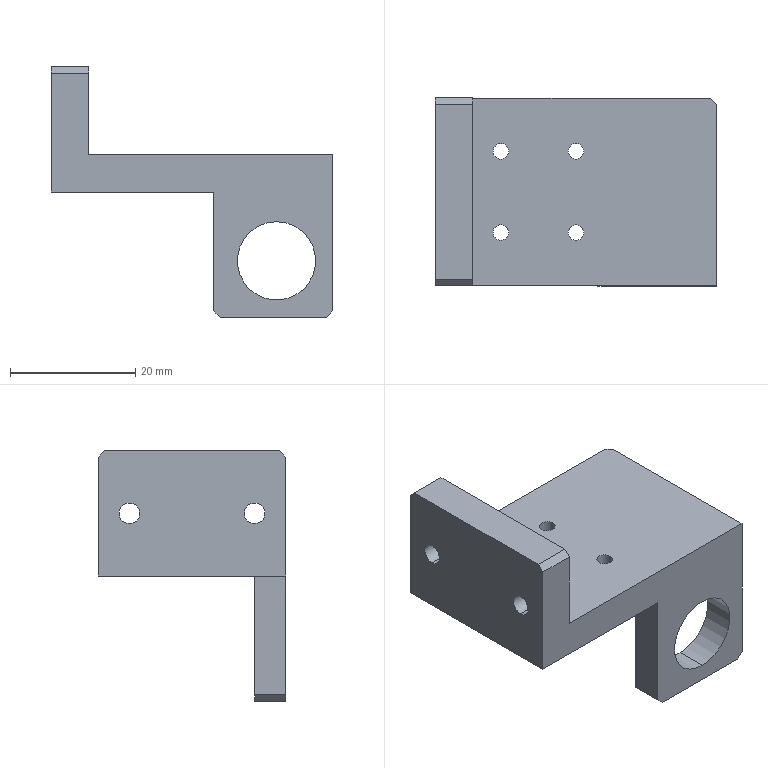Component | SolidWorks | F01AE00111-A5211-1 | 1 solid | 34 faces | box 45 x 30 x 40 mm | volume 11634 mm3 | cylinder 16 | plane 16 | cone 2 | commonest cylinder face diameters 2.5 x10 3.3 x4 12.5 x2
build123d program:
from build123d import *

# Parameters (mm, degrees)
SKETCH1_W             = 45
SKETCH1_H             = 30
BOSS_EXTRUDE1_DEPTH   = 3
SKETCH3_W             = 6
SKETCH3_H             = 30
BOSS_EXTRUDE3_DEPTH   = 14
M4_TAPPED_HOLE1_D     = 3.3
M4_TAPPED_HOLE1_DEPTH = 10.1
M4_TAPPED_HOLE1_TIP   = 0.9914
SKETCH9_W             = 19
SKETCH9_H             = 5
BOSS_EXTRUDE4_DEPTH   = 20
SKETCH10_R            = 6.25
CUT_EXTRUDE2_DEPTH    = 41.746
CHAMFER1_SIZE         = 1
SKETCH11_R            = 1.25
CUT_EXTRUDE3_DEPTH    = 38.513
M3_TAPPED_HOLE1_D     = 2.5
M3_TAPPED_HOLE1_DEPTH = 7.5
M3_TAPPED_HOLE1_TIP   = 0.7511


with BuildPart() as part:
    # Sketch1 → Boss-Extrude1 (new, symmetric)
    with BuildSketch(Plane.XY):
        Rectangle(SKETCH1_W, SKETCH1_H)
    extrude(amount=BOSS_EXTRUDE1_DEPTH, both=True)

    # Sketch3 → Boss-Extrude3 (add)
    with BuildSketch(Plane.XY.offset(3)):
        with Locations((-19.5, 0)):
            Rectangle(SKETCH3_W, SKETCH3_H)
    extrude(amount=BOSS_EXTRUDE3_DEPTH)

    # M4 Tapped Hole1
    with Locations(Plane.ZY.offset(22.5)):
        with Locations((7, -10), (7, 10)):
            Hole(M4_TAPPED_HOLE1_D / 2, depth=M4_TAPPED_HOLE1_DEPTH)
            with Locations((0, 0, -(M4_TAPPED_HOLE1_DEPTH + M4_TAPPED_HOLE1_TIP / 2))):  # 118° drill point
                Cone(0, M4_TAPPED_HOLE1_D / 2, M4_TAPPED_HOLE1_TIP, mode=Mode.SUBTRACT)

    # Sketch9 → Boss-Extrude4 (add)
    with BuildSketch(Plane(origin=(0, 0, -3), x_dir=(-1, 0, 0), z_dir=(0, 0, -1))):
        with Locations((-13, -12.5)):
            Rectangle(SKETCH9_W, SKETCH9_H)
    extrude(amount=BOSS_EXTRUDE4_DEPTH)

    # Sketch10 → Cut-Extrude2 (cut, through all)
    with BuildSketch(Plane(origin=(0, -10, 0), x_dir=(-1, 0, 0), z_dir=(0, 1, 0))):
        with Locations(Location((-13.5, -14, 0), (0, 0, 90))):
            Circle(SKETCH10_R)
    extrude(amount=-CUT_EXTRUDE2_DEPTH, mode=Mode.SUBTRACT)

    # Chamfer1
    chamfer1_edges = [part.edges().sort_by_distance(p)[0] for p in [
        (-19.5, -15, 17),
        (-19.5, 15, 17),
        (22.5, 15, 0),
        (22.5, -12.5, -23),
        (3.5, -12.5, -23),
    ]]
    chamfer(chamfer1_edges, length=CHAMFER1_SIZE)

    # Sketch11 → Cut-Extrude3 (cut, through all)
    with BuildSketch(Plane.XY.offset(3)):
        with Locations((-12, 6.5)):
            Circle(SKETCH11_R)
        with Locations((0, 6.5)):
            Circle(SKETCH11_R)
        with Locations((-12, -6.5)):
            Circle(SKETCH11_R)
        with Locations((0, -6.5)):
            Circle(SKETCH11_R)
    extrude(amount=-CUT_EXTRUDE3_DEPTH, mode=Mode.SUBTRACT)

    # M3 Tapped Hole1
    with Locations(Plane(origin=(0, 0, -23), x_dir=(-1, 0, 0), z_dir=(0, 0, -1))):
        with Locations((-6.5, -12.5)):
            Hole(M3_TAPPED_HOLE1_D / 2, depth=M3_TAPPED_HOLE1_DEPTH)
            with Locations((0, 0, -(M3_TAPPED_HOLE1_DEPTH + M3_TAPPED_HOLE1_TIP / 2))):  # 118° drill point
                Cone(0, M3_TAPPED_HOLE1_D / 2, M3_TAPPED_HOLE1_TIP, mode=Mode.SUBTRACT)


solid = part.part

# Placed as in the assembly
solid = solid.moved(Location((-57.681, -35.188, -297.979), (0, 0, 0)))